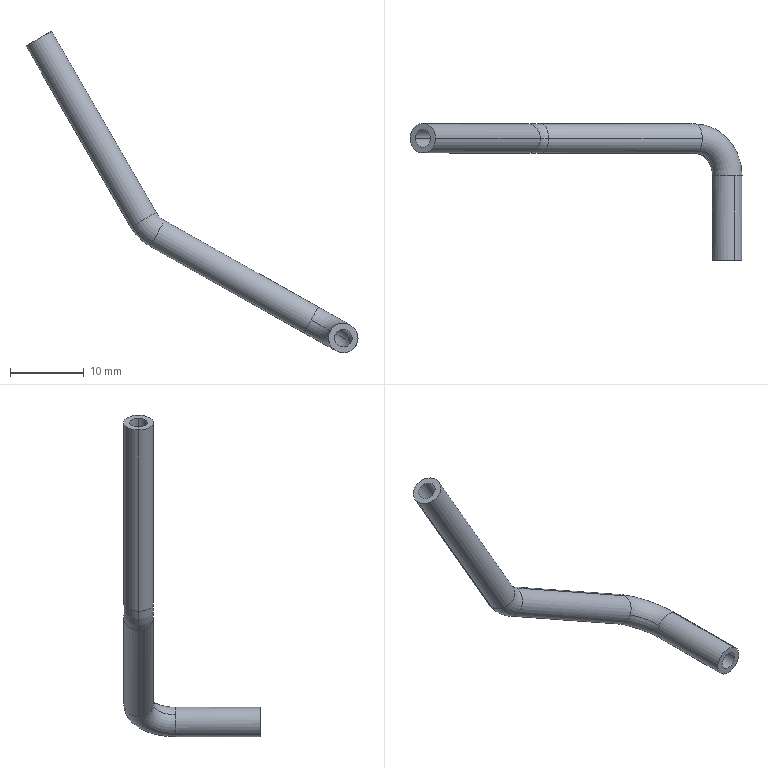Component | SolidWorks | WaterPipe2-1 | 1 solid | 22 faces | box 44.91 x 18.45 x 43.5 mm | volume 596 mm3 | cylinder 12 | torus 8 | plane 2 | commonest cylinder face diameters 2.4 x6 4 x6
build123d program:
from build123d import *

# Parameters (mm, degrees)
SCAN_THIN_FEATURE1_PROFILE_R   = 2
SCAN_THIN_FEATURE1_PROFILE_R_2 = 1.2


with BuildPart() as part:
    # Scan-Thin Feature1: sweep along a curve in space
    with BuildLine() as scan_thin_feature1_path:
        Line((0, -15.405, 0), (0, -3.951, 0))
        ThreePointArc((-5, 1.049, 0), (-1.464, -0.4154, 0), (0, -3.951, 0))
        Line((-5, 1.049, 0), (-28.841, 1.049, 0))
        ThreePointArc((-31.391, 1.049, 0.6989), (-30.163, 1.049, 0.1779), (-28.841, 1.049, 0))
        Line((-31.391, 1.049, 0.6989), (-55.737, 1.049, 15.131))
    # Scan-Thin Feature1 profile (on start of the path) → Scan-Thin Feature1 (sweep)
    with BuildSketch(Plane.ZX.offset(-15.405)):
        Circle(SCAN_THIN_FEATURE1_PROFILE_R)
        Circle(SCAN_THIN_FEATURE1_PROFILE_R_2, mode=Mode.SUBTRACT)
    sweep(path=scan_thin_feature1_path.line)


solid = part.part

# Placed as in the assembly
solid = solid.moved(Location((-15.981, 32.512, 80), (0, 29.34, 0)))
STEP:
#1=COLOUR_RGB('',0.7922,0.8196,0.9333);
#2=FILL_AREA_STYLE_COLOUR('',#1);
#3=FILL_AREA_STYLE('',(#2));
#4=SURFACE_STYLE_FILL_AREA(#3);
#5=SURFACE_SIDE_STYLE('',(#4));
#6=SURFACE_STYLE_USAGE(.BOTH.,#5);
#7=PRESENTATION_STYLE_ASSIGNMENT((#6));
#8=CARTESIAN_POINT('',(-1.596,1.321,3.747));
#9=VERTEX_POINT('',#8);
#10=CARTESIAN_POINT('',(-1.642,1.321,3.665));
#11=VERTEX_POINT('',#10);
#12=CARTESIAN_POINT('',(-1.619,1.321,3.706));
#13=DIRECTION('',(0.8717,-0.,-0.49));
#14=DIRECTION('',(0.49,-0.,0.8717));
#15=AXIS2_PLACEMENT_3D('',#12,#13,#14);
#16=CIRCLE('',#15,0.04724);
#17=EDGE_CURVE('',#9,#11,#16,.T.);
#18=ORIENTED_EDGE('',*,*,#17,.T.);
#19=CARTESIAN_POINT('',(-1.734,1.321,3.756));
#20=VERTEX_POINT('',#19);
#21=CARTESIAN_POINT('',(-1.523,1.321,3.878));
#22=DIRECTION('',(-0.,1.,-0.));
#23=DIRECTION('',(0.,0.,1.));
#24=AXIS2_PLACEMENT_3D('',#21,#22,#23);
#25=CIRCLE('',#24,0.2441);
#26=EDGE_CURVE('',#11,#20,#25,.T.);
#27=ORIENTED_EDGE('',*,*,#26,.T.);
#28=CARTESIAN_POINT('',(-1.652,1.321,3.803));
#29=VERTEX_POINT('',#28);
#30=CARTESIAN_POINT('',(-1.693,1.321,3.779));
#31=DIRECTION('',(0.5,-0.,-0.866));
#32=DIRECTION('',(-0.866,0.,-0.5));
#33=AXIS2_PLACEMENT_3D('',#30,#31,#32);
#34=CIRCLE('',#33,0.04724);
#35=EDGE_CURVE('',#29,#20,#34,.T.);
#36=ORIENTED_EDGE('',*,*,#35,.F.);
#37=CARTESIAN_POINT('',(-1.523,1.321,3.878));
#38=DIRECTION('',(-0.,1.,-0.));
#39=DIRECTION('',(0.,0.,1.));
#40=AXIS2_PLACEMENT_3D('',#37,#38,#39);
#41=CIRCLE('',#40,0.1496);
#42=EDGE_CURVE('',#9,#29,#41,.T.);
#43=ORIENTED_EDGE('',*,*,#42,.F.);
#44=EDGE_LOOP('',(#18,#27,#36,#43));
#45=FACE_OUTER_BOUND('',#44,.T.);
#46=CARTESIAN_POINT('',(-1.523,1.321,3.878));
#47=DIRECTION('',(-0.,1.,-0.));
#48=DIRECTION('',(0.49,0.,0.8717));
#49=AXIS2_PLACEMENT_3D('',#46,#47,#48);
#50=TOROIDAL_SURFACE('',#49,0.1969,0.04724);
#51=ADVANCED_FACE('',(#45),#50,.F.);
#52=CARTESIAN_POINT('',(-0.6523,1.124,3.108));
#53=VERTEX_POINT('',#52);
#54=CARTESIAN_POINT('',(-0.588,1.124,3.126));
#55=VERTEX_POINT('',#54);
#56=CARTESIAN_POINT('',(-0.6292,1.124,3.15));
#57=DIRECTION('',(0.,-1.,0.));
#58=DIRECTION('',(0.49,0.,0.8717));
#59=AXIS2_PLACEMENT_3D('',#56,#57,#58);
#60=CIRCLE('',#59,0.04724);
#61=EDGE_CURVE('',#53,#55,#60,.T.);
#62=ORIENTED_EDGE('',*,*,#61,.T.);
#63=CARTESIAN_POINT('',(-0.8008,1.369,3.246));
#64=VERTEX_POINT('',#63);
#65=CARTESIAN_POINT('',(-0.8008,1.124,3.246));
#66=DIRECTION('',(0.49,0.,0.8717));
#67=DIRECTION('',(0.8717,0.,-0.49));
#68=AXIS2_PLACEMENT_3D('',#65,#66,#67);
#69=CIRCLE('',#68,0.2441);
#70=EDGE_CURVE('',#55,#64,#69,.T.);
#71=ORIENTED_EDGE('',*,*,#70,.T.);
#72=CARTESIAN_POINT('',(-0.8239,1.321,3.205));
#73=VERTEX_POINT('',#72);
#74=CARTESIAN_POINT('',(-0.8008,1.321,3.246));
#75=DIRECTION('',(0.8717,0.,-0.49));
#76=DIRECTION('',(-0.,1.,0.));
#77=AXIS2_PLACEMENT_3D('',#74,#75,#76);
#78=CIRCLE('',#77,0.04724);
#79=EDGE_CURVE('',#73,#64,#78,.T.);
#80=ORIENTED_EDGE('',*,*,#79,.F.);
#81=CARTESIAN_POINT('',(-0.8008,1.274,3.246));
#82=VERTEX_POINT('',#81);
#83=CARTESIAN_POINT('',(-0.8008,1.321,3.246));
#84=DIRECTION('',(0.8717,0.,-0.49));
#85=DIRECTION('',(-0.,1.,0.));
#86=AXIS2_PLACEMENT_3D('',#83,#84,#85);
#87=CIRCLE('',#86,0.04724);
#88=EDGE_CURVE('',#82,#73,#87,.T.);
#89=ORIENTED_EDGE('',*,*,#88,.F.);
#90=CARTESIAN_POINT('',(-0.6704,1.124,3.173));
#91=VERTEX_POINT('',#90);
#92=CARTESIAN_POINT('',(-0.8008,1.124,3.246));
#93=DIRECTION('',(0.49,0.,0.8717));
#94=DIRECTION('',(0.8717,0.,-0.49));
#95=AXIS2_PLACEMENT_3D('',#92,#93,#94);
#96=CIRCLE('',#95,0.1496);
#97=EDGE_CURVE('',#91,#82,#96,.T.);
#98=ORIENTED_EDGE('',*,*,#97,.F.);
#99=CARTESIAN_POINT('',(-0.6292,1.124,3.15));
#100=DIRECTION('',(0.,-1.,0.));
#101=DIRECTION('',(0.49,0.,0.8717));
#102=AXIS2_PLACEMENT_3D('',#99,#100,#101);
#103=CIRCLE('',#102,0.04724);
#104=EDGE_CURVE('',#91,#53,#103,.T.);
#105=ORIENTED_EDGE('',*,*,#104,.T.);
#106=EDGE_LOOP('',(#62,#71,#80,#89,#98,#105));
#107=FACE_OUTER_BOUND('',#106,.T.);
#108=CARTESIAN_POINT('',(-0.8008,1.124,3.246));
#109=DIRECTION('',(0.49,0.,0.8717));
#110=DIRECTION('',(0.8717,0.,-0.49));
#111=AXIS2_PLACEMENT_3D('',#108,#109,#110);
#112=TOROIDAL_SURFACE('',#111,0.1969,0.04724);
#113=ADVANCED_FACE('',(#107),#112,.F.);
#114=CARTESIAN_POINT('',(-1.658,1.321,3.637));
#115=VERTEX_POINT('',#114);
#116=CARTESIAN_POINT('',(-1.58,1.321,3.775));
#117=VERTEX_POINT('',#116);
#118=CARTESIAN_POINT('',(-1.619,1.321,3.706));
#119=DIRECTION('',(0.8717,-0.,-0.49));
#120=DIRECTION('',(-0.49,0.,-0.8717));
#121=AXIS2_PLACEMENT_3D('',#118,#119,#120);
#122=CIRCLE('',#121,0.07874);
#123=EDGE_CURVE('',#115,#117,#122,.T.);
#124=ORIENTED_EDGE('',*,*,#123,.F.);
#125=CARTESIAN_POINT('',(-1.761,1.321,3.74));
#126=VERTEX_POINT('',#125);
#127=CARTESIAN_POINT('',(-1.523,1.321,3.878));
#128=DIRECTION('',(-0.,1.,-0.));
#129=DIRECTION('',(0.,0.,1.));
#130=AXIS2_PLACEMENT_3D('',#127,#128,#129);
#131=CIRCLE('',#130,0.2756);
#132=EDGE_CURVE('',#115,#126,#131,.T.);
#133=ORIENTED_EDGE('',*,*,#132,.T.);
#134=CARTESIAN_POINT('',(-1.625,1.321,3.819));
#135=VERTEX_POINT('',#134);
#136=CARTESIAN_POINT('',(-1.693,1.321,3.779));
#137=DIRECTION('',(0.5,-0.,-0.866));
#138=DIRECTION('',(-0.866,0.,-0.5));
#139=AXIS2_PLACEMENT_3D('',#136,#137,#138);
#140=CIRCLE('',#139,0.07874);
#141=EDGE_CURVE('',#126,#135,#140,.T.);
#142=ORIENTED_EDGE('',*,*,#141,.T.);
#143=CARTESIAN_POINT('',(-1.523,1.321,3.878));
#144=DIRECTION('',(-0.,1.,-0.));
#145=DIRECTION('',(0.,0.,1.));
#146=AXIS2_PLACEMENT_3D('',#143,#144,#145);
#147=CIRCLE('',#146,0.1181);
#148=EDGE_CURVE('',#117,#135,#147,.T.);
#149=ORIENTED_EDGE('',*,*,#148,.F.);
#150=EDGE_LOOP('',(#124,#133,#142,#149));
#151=FACE_OUTER_BOUND('',#150,.T.);
#152=CARTESIAN_POINT('',(-1.523,1.321,3.878));
#153=DIRECTION('',(-0.,1.,-0.));
#154=DIRECTION('',(0.49,0.,0.8717));
#155=AXIS2_PLACEMENT_3D('',#152,#153,#154);
#156=TOROIDAL_SURFACE('',#155,0.1969,0.07874);
#157=ADVANCED_FACE('',(#151),#156,.T.);
#158=CARTESIAN_POINT('',(-0.5605,1.124,3.111));
#159=VERTEX_POINT('',#158);
#160=CARTESIAN_POINT('',(-0.5906,1.124,3.218));
#161=VERTEX_POINT('',#160);
#162=CARTESIAN_POINT('',(-0.6292,1.124,3.15));
#163=DIRECTION('',(-0.,-1.,-0.));
#164=DIRECTION('',(-0.49,0.,-0.8717));
#165=AXIS2_PLACEMENT_3D('',#162,#163,#164);
#166=CIRCLE('',#165,0.07874);
#167=EDGE_CURVE('',#159,#161,#166,.T.);
#168=ORIENTED_EDGE('',*,*,#167,.F.);
#169=CARTESIAN_POINT('',(-0.8008,1.4,3.246));
#170=VERTEX_POINT('',#169);
#171=CARTESIAN_POINT('',(-0.8008,1.124,3.246));
#172=DIRECTION('',(0.49,0.,0.8717));
#173=DIRECTION('',(0.8717,0.,-0.49));
#174=AXIS2_PLACEMENT_3D('',#171,#172,#173);
#175=CIRCLE('',#174,0.2756);
#176=EDGE_CURVE('',#159,#170,#175,.T.);
#177=ORIENTED_EDGE('',*,*,#176,.T.);
#178=CARTESIAN_POINT('',(-0.7622,1.321,3.315));
#179=VERTEX_POINT('',#178);
#180=CARTESIAN_POINT('',(-0.8008,1.321,3.246));
#181=DIRECTION('',(0.8717,-0.,-0.49));
#182=DIRECTION('',(-0.49,0.,-0.8717));
#183=AXIS2_PLACEMENT_3D('',#180,#181,#182);
#184=CIRCLE('',#183,0.07874);
#185=EDGE_CURVE('',#170,#179,#184,.T.);
#186=ORIENTED_EDGE('',*,*,#185,.T.);
#187=CARTESIAN_POINT('',(-0.8008,1.243,3.246));
#188=VERTEX_POINT('',#187);
#189=CARTESIAN_POINT('',(-0.8008,1.321,3.246));
#190=DIRECTION('',(0.8717,-0.,-0.49));
#191=DIRECTION('',(-0.49,0.,-0.8717));
#192=AXIS2_PLACEMENT_3D('',#189,#190,#191);
#193=CIRCLE('',#192,0.07874);
#194=EDGE_CURVE('',#179,#188,#193,.T.);
#195=ORIENTED_EDGE('',*,*,#194,.T.);
#196=CARTESIAN_POINT('',(-0.6978,1.124,3.188));
#197=VERTEX_POINT('',#196);
#198=CARTESIAN_POINT('',(-0.8008,1.124,3.246));
#199=DIRECTION('',(0.49,0.,0.8717));
#200=DIRECTION('',(0.8717,0.,-0.49));
#201=AXIS2_PLACEMENT_3D('',#198,#199,#200);
#202=CIRCLE('',#201,0.1181);
#203=EDGE_CURVE('',#197,#188,#202,.T.);
#204=ORIENTED_EDGE('',*,*,#203,.F.);
#205=CARTESIAN_POINT('',(-0.6292,1.124,3.15));
#206=DIRECTION('',(-0.,-1.,-0.));
#207=DIRECTION('',(-0.49,0.,-0.8717));
#208=AXIS2_PLACEMENT_3D('',#205,#206,#207);
#209=CIRCLE('',#208,0.07874);
#210=EDGE_CURVE('',#161,#197,#209,.T.);
#211=ORIENTED_EDGE('',*,*,#210,.F.);
#212=EDGE_LOOP('',(#168,#177,#186,#195,#204,#211));
#213=FACE_OUTER_BOUND('',#212,.T.);
#214=CARTESIAN_POINT('',(-0.8008,1.124,3.246));
#215=DIRECTION('',(0.49,0.,0.8717));
#216=DIRECTION('',(0.8717,0.,-0.49));
#217=AXIS2_PLACEMENT_3D('',#214,#215,#216);
#218=TOROIDAL_SURFACE('',#217,0.1969,0.07874);
#219=ADVANCED_FACE('',(#213),#218,.T.);
#220=ORIENTED_EDGE('',*,*,#35,.T.);
#221=CARTESIAN_POINT('',(-2.291,1.321,4.721));
#222=VERTEX_POINT('',#221);
#223=CARTESIAN_POINT('',(-1.734,1.321,3.756));
#224=DIRECTION('',(-0.5,0.,0.866));
#225=VECTOR('',#224,39.37);
#226=LINE('',#223,#225);
#227=EDGE_CURVE('',#20,#222,#226,.T.);
#228=ORIENTED_EDGE('',*,*,#227,.T.);
#229=CARTESIAN_POINT('',(-2.209,1.321,4.768));
#230=VERTEX_POINT('',#229);
#231=CARTESIAN_POINT('',(-2.25,1.321,4.744));
#232=DIRECTION('',(0.5,-0.,-0.866));
#233=DIRECTION('',(-0.866,0.,-0.5));
#234=AXIS2_PLACEMENT_3D('',#231,#232,#233);
#235=CIRCLE('',#234,0.04724);
#236=EDGE_CURVE('',#230,#222,#235,.T.);
#237=ORIENTED_EDGE('',*,*,#236,.F.);
#238=CARTESIAN_POINT('',(-1.652,1.321,3.803));
#239=DIRECTION('',(-0.5,0.,0.866));
#240=VECTOR('',#239,39.37);
#241=LINE('',#238,#240);
#242=EDGE_CURVE('',#29,#230,#241,.T.);
#243=ORIENTED_EDGE('',*,*,#242,.F.);
#244=EDGE_LOOP('',(#220,#228,#237,#243));
#245=FACE_OUTER_BOUND('',#244,.T.);
#246=CARTESIAN_POINT('',(-1.693,1.321,3.779));
#247=DIRECTION('',(-0.5,0.,0.866));
#248=DIRECTION('',(0.866,0.,0.5));
#249=AXIS2_PLACEMENT_3D('',#246,#247,#248);
#250=CYLINDRICAL_SURFACE('',#249,0.04724);
#251=ADVANCED_FACE('',(#245),#250,.F.);
#252=CARTESIAN_POINT('',(-0.7776,1.321,3.287));
#253=VERTEX_POINT('',#252);
#254=CARTESIAN_POINT('',(-0.8008,1.321,3.246));
#255=DIRECTION('',(0.8717,0.,-0.49));
#256=DIRECTION('',(-0.,1.,0.));
#257=AXIS2_PLACEMENT_3D('',#254,#255,#256);
#258=CIRCLE('',#257,0.04724);
#259=EDGE_CURVE('',#253,#82,#258,.T.);
#260=ORIENTED_EDGE('',*,*,#259,.T.);
#261=ORIENTED_EDGE('',*,*,#88,.T.);
#262=CARTESIAN_POINT('',(-0.8239,1.321,3.205));
#263=DIRECTION('',(-0.8717,0.,0.49));
#264=VECTOR('',#263,39.37);
#265=LINE('',#262,#264);
#266=EDGE_CURVE('',#73,#11,#265,.T.);
#267=ORIENTED_EDGE('',*,*,#266,.T.);
#268=ORIENTED_EDGE('',*,*,#17,.F.);
#269=CARTESIAN_POINT('',(-0.7776,1.321,3.287));
#270=DIRECTION('',(-0.8717,0.,0.49));
#271=VECTOR('',#270,39.37);
#272=LINE('',#269,#271);
#273=EDGE_CURVE('',#253,#9,#272,.T.);
#274=ORIENTED_EDGE('',*,*,#273,.F.);
#275=EDGE_LOOP('',(#260,#261,#267,#268,#274));
#276=FACE_OUTER_BOUND('',#275,.T.);
#277=CARTESIAN_POINT('',(-0.8008,1.321,3.246));
#278=DIRECTION('',(-0.8717,0.,0.49));
#279=DIRECTION('',(0.49,0.,0.8717));
#280=AXIS2_PLACEMENT_3D('',#277,#278,#279);
#281=CYLINDRICAL_SURFACE('',#280,0.04724);
#282=ADVANCED_FACE('',(#276),#281,.F.);
#283=CARTESIAN_POINT('',(-0.606,0.6735,3.191));
#284=VERTEX_POINT('',#283);
#285=CARTESIAN_POINT('',(-0.6523,0.6735,3.108));
#286=VERTEX_POINT('',#285);
#287=CARTESIAN_POINT('',(-0.6292,0.6735,3.15));
#288=DIRECTION('',(-0.,-1.,-0.));
#289=DIRECTION('',(-0.49,0.,-0.8717));
#290=AXIS2_PLACEMENT_3D('',#287,#288,#289);
#291=CIRCLE('',#290,0.04724);
#292=EDGE_CURVE('',#284,#286,#291,.T.);
#293=ORIENTED_EDGE('',*,*,#292,.T.);
#294=CARTESIAN_POINT('',(-0.6523,0.6735,3.108));
#295=DIRECTION('',(-0.,1.,-0.));
#296=VECTOR('',#295,39.37);
#297=LINE('',#294,#296);
#298=EDGE_CURVE('',#286,#53,#297,.T.);
#299=ORIENTED_EDGE('',*,*,#298,.T.);
#300=ORIENTED_EDGE('',*,*,#104,.F.);
#301=CARTESIAN_POINT('',(-0.606,1.124,3.191));
#302=VERTEX_POINT('',#301);
#303=CARTESIAN_POINT('',(-0.6292,1.124,3.15));
#304=DIRECTION('',(0.,-1.,0.));
#305=DIRECTION('',(0.49,0.,0.8717));
#306=AXIS2_PLACEMENT_3D('',#303,#304,#305);
#307=CIRCLE('',#306,0.04724);
#308=EDGE_CURVE('',#302,#91,#307,.T.);
#309=ORIENTED_EDGE('',*,*,#308,.F.);
#310=CARTESIAN_POINT('',(-0.606,0.6735,3.191));
#311=DIRECTION('',(-0.,1.,-0.));
#312=VECTOR('',#311,39.37);
#313=LINE('',#310,#312);
#314=EDGE_CURVE('',#284,#302,#313,.T.);
#315=ORIENTED_EDGE('',*,*,#314,.F.);
#316=EDGE_LOOP('',(#293,#299,#300,#309,#315));
#317=FACE_OUTER_BOUND('',#316,.T.);
#318=CARTESIAN_POINT('',(-0.6292,0.6735,3.15));
#319=DIRECTION('',(-0.,1.,-0.));
#320=DIRECTION('',(0.49,0.,0.8717));
#321=AXIS2_PLACEMENT_3D('',#318,#319,#320);
#322=CYLINDRICAL_SURFACE('',#321,0.04724);
#323=ADVANCED_FACE('',(#317),#322,.F.);
#324=ORIENTED_EDGE('',*,*,#141,.F.);
#325=CARTESIAN_POINT('',(-2.318,1.321,4.705));
#326=VERTEX_POINT('',#325);
#327=CARTESIAN_POINT('',(-1.761,1.321,3.74));
#328=DIRECTION('',(-0.5,0.,0.866));
#329=VECTOR('',#328,39.37);
#330=LINE('',#327,#329);
#331=EDGE_CURVE('',#126,#326,#330,.T.);
#332=ORIENTED_EDGE('',*,*,#331,.T.);
#333=CARTESIAN_POINT('',(-2.182,1.321,4.784));
#334=VERTEX_POINT('',#333);
#335=CARTESIAN_POINT('',(-2.25,1.321,4.744));
#336=DIRECTION('',(0.5,-0.,-0.866));
#337=DIRECTION('',(-0.866,0.,-0.5));
#338=AXIS2_PLACEMENT_3D('',#335,#336,#337);
#339=CIRCLE('',#338,0.07874);
#340=EDGE_CURVE('',#326,#334,#339,.T.);
#341=ORIENTED_EDGE('',*,*,#340,.T.);
#342=CARTESIAN_POINT('',(-1.625,1.321,3.819));
#343=DIRECTION('',(-0.5,0.,0.866));
#344=VECTOR('',#343,39.37);
#345=LINE('',#342,#344);
#346=EDGE_CURVE('',#135,#334,#345,.T.);
#347=ORIENTED_EDGE('',*,*,#346,.F.);
#348=EDGE_LOOP('',(#324,#332,#341,#347));
#349=FACE_OUTER_BOUND('',#348,.T.);
#350=CARTESIAN_POINT('',(-1.693,1.321,3.779));
#351=DIRECTION('',(-0.5,0.,0.866));
#352=DIRECTION('',(0.866,0.,0.5));
#353=AXIS2_PLACEMENT_3D('',#350,#351,#352);
#354=CYLINDRICAL_SURFACE('',#353,0.07874);
#355=ADVANCED_FACE('',(#349),#354,.T.);
#356=CARTESIAN_POINT('',(-0.8394,1.321,3.177));
#357=VERTEX_POINT('',#356);
#358=CARTESIAN_POINT('',(-0.8008,1.321,3.246));
#359=DIRECTION('',(0.8717,-0.,-0.49));
#360=DIRECTION('',(-0.49,0.,-0.8717));
#361=AXIS2_PLACEMENT_3D('',#358,#359,#360);
#362=CIRCLE('',#361,0.07874);
#363=EDGE_CURVE('',#357,#170,#362,.T.);
#364=ORIENTED_EDGE('',*,*,#363,.F.);
#365=CARTESIAN_POINT('',(-0.8394,1.321,3.177));
#366=DIRECTION('',(-0.8717,0.,0.49));
#367=VECTOR('',#366,39.37);
#368=LINE('',#365,#367);
#369=EDGE_CURVE('',#357,#115,#368,.T.);
#370=ORIENTED_EDGE('',*,*,#369,.T.);
#371=ORIENTED_EDGE('',*,*,#123,.T.);
#372=CARTESIAN_POINT('',(-0.7622,1.321,3.315));
#373=DIRECTION('',(-0.8717,0.,0.49));
#374=VECTOR('',#373,39.37);
#375=LINE('',#372,#374);
#376=EDGE_CURVE('',#179,#117,#375,.T.);
#377=ORIENTED_EDGE('',*,*,#376,.F.);
#378=ORIENTED_EDGE('',*,*,#185,.F.);
#379=EDGE_LOOP('',(#364,#370,#371,#377,#378));
#380=FACE_OUTER_BOUND('',#379,.T.);
#381=CARTESIAN_POINT('',(-0.8008,1.321,3.246));
#382=DIRECTION('',(-0.8717,0.,0.49));
#383=DIRECTION('',(0.49,0.,0.8717));
#384=AXIS2_PLACEMENT_3D('',#381,#382,#383);
#385=CYLINDRICAL_SURFACE('',#384,0.07874);
#386=ADVANCED_FACE('',(#380),#385,.T.);
#387=CARTESIAN_POINT('',(-0.6678,0.6735,3.081));
#388=VERTEX_POINT('',#387);
#389=CARTESIAN_POINT('',(-0.5906,0.6735,3.218));
#390=VERTEX_POINT('',#389);
#391=CARTESIAN_POINT('',(-0.6292,0.6735,3.15));
#392=DIRECTION('',(-0.,-1.,-0.));
#393=DIRECTION('',(-0.49,0.,-0.8717));
#394=AXIS2_PLACEMENT_3D('',#391,#392,#393);
#395=CIRCLE('',#394,0.07874);
#396=EDGE_CURVE('',#388,#390,#395,.T.);
#397=ORIENTED_EDGE('',*,*,#396,.F.);
#398=CARTESIAN_POINT('',(-0.6678,1.124,3.081));
#399=VERTEX_POINT('',#398);
#400=CARTESIAN_POINT('',(-0.6678,0.6735,3.081));
#401=DIRECTION('',(-0.,1.,-0.));
#402=VECTOR('',#401,39.37);
#403=LINE('',#400,#402);
#404=EDGE_CURVE('',#388,#399,#403,.T.);
#405=ORIENTED_EDGE('',*,*,#404,.T.);
#406=CARTESIAN_POINT('',(-0.6292,1.124,3.15));
#407=DIRECTION('',(-0.,-1.,-0.));
#408=DIRECTION('',(-0.49,0.,-0.8717));
#409=AXIS2_PLACEMENT_3D('',#406,#407,#408);
#410=CIRCLE('',#409,0.07874);
#411=EDGE_CURVE('',#399,#159,#410,.T.);
#412=ORIENTED_EDGE('',*,*,#411,.T.);
#413=ORIENTED_EDGE('',*,*,#167,.T.);
#414=CARTESIAN_POINT('',(-0.5906,0.6735,3.218));
#415=DIRECTION('',(-0.,1.,-0.));
#416=VECTOR('',#415,39.37);
#417=LINE('',#414,#416);
#418=EDGE_CURVE('',#390,#161,#417,.T.);
#419=ORIENTED_EDGE('',*,*,#418,.F.);
#420=EDGE_LOOP('',(#397,#405,#412,#413,#419));
#421=FACE_OUTER_BOUND('',#420,.T.);
#422=CARTESIAN_POINT('',(-0.6292,0.6735,3.15));
#423=DIRECTION('',(-0.,1.,-0.));
#424=DIRECTION('',(0.49,0.,0.8717));
#425=AXIS2_PLACEMENT_3D('',#422,#423,#424);
#426=CYLINDRICAL_SURFACE('',#425,0.07874);
#427=ADVANCED_FACE('',(#421),#426,.T.);
#428=ORIENTED_EDGE('',*,*,#331,.F.);
#429=CARTESIAN_POINT('',(-1.693,1.321,3.779));
#430=DIRECTION('',(0.5,-0.,-0.866));
#431=DIRECTION('',(-0.866,0.,-0.5));
#432=AXIS2_PLACEMENT_3D('',#429,#430,#431);
#433=CIRCLE('',#432,0.07874);
#434=EDGE_CURVE('',#135,#126,#433,.T.);
#435=ORIENTED_EDGE('',*,*,#434,.F.);
#436=ORIENTED_EDGE('',*,*,#346,.T.);
#437=CARTESIAN_POINT('',(-2.25,1.321,4.744));
#438=DIRECTION('',(0.5,-0.,-0.866));
#439=DIRECTION('',(-0.866,0.,-0.5));
#440=AXIS2_PLACEMENT_3D('',#437,#438,#439);
#441=CIRCLE('',#440,0.07874);
#442=EDGE_CURVE('',#334,#326,#441,.T.);
#443=ORIENTED_EDGE('',*,*,#442,.T.);
#444=EDGE_LOOP('',(#428,#435,#436,#443));
#445=FACE_OUTER_BOUND('',#444,.T.);
#446=CARTESIAN_POINT('',(-1.693,1.321,3.779));
#447=DIRECTION('',(-0.5,0.,0.866));
#448=DIRECTION('',(0.866,0.,0.5));
#449=AXIS2_PLACEMENT_3D('',#446,#447,#448);
#450=CYLINDRICAL_SURFACE('',#449,0.07874);
#451=ADVANCED_FACE('',(#445),#450,.T.);
#452=ORIENTED_EDGE('',*,*,#132,.F.);
#453=CARTESIAN_POINT('',(-1.619,1.321,3.706));
#454=DIRECTION('',(0.8717,-0.,-0.49));
#455=DIRECTION('',(-0.49,0.,-0.8717));
#456=AXIS2_PLACEMENT_3D('',#453,#454,#455);
#457=CIRCLE('',#456,0.07874);
#458=EDGE_CURVE('',#117,#115,#457,.T.);
#459=ORIENTED_EDGE('',*,*,#458,.F.);
#460=ORIENTED_EDGE('',*,*,#148,.T.);
#461=ORIENTED_EDGE('',*,*,#434,.T.);
#462=EDGE_LOOP('',(#452,#459,#460,#461));
#463=FACE_OUTER_BOUND('',#462,.T.);
#464=CARTESIAN_POINT('',(-1.523,1.321,3.878));
#465=DIRECTION('',(-0.,1.,-0.));
#466=DIRECTION('',(0.49,0.,0.8717));
#467=AXIS2_PLACEMENT_3D('',#464,#465,#466);
#468=TOROIDAL_SURFACE('',#467,0.1969,0.07874);
#469=ADVANCED_FACE('',(#463),#468,.T.);
#470=ORIENTED_EDGE('',*,*,#369,.F.);
#471=CARTESIAN_POINT('',(-0.8008,1.321,3.246));
#472=DIRECTION('',(0.8717,-0.,-0.49));
#473=DIRECTION('',(-0.49,0.,-0.8717));
#474=AXIS2_PLACEMENT_3D('',#471,#472,#473);
#475=CIRCLE('',#474,0.07874);
#476=EDGE_CURVE('',#188,#357,#475,.T.);
#477=ORIENTED_EDGE('',*,*,#476,.F.);
#478=ORIENTED_EDGE('',*,*,#194,.F.);
#479=ORIENTED_EDGE('',*,*,#376,.T.);
#480=ORIENTED_EDGE('',*,*,#458,.T.);
#481=EDGE_LOOP('',(#470,#477,#478,#479,#480));
#482=FACE_OUTER_BOUND('',#481,.T.);
#483=CARTESIAN_POINT('',(-0.8008,1.321,3.246));
#484=DIRECTION('',(-0.8717,0.,0.49));
#485=DIRECTION('',(0.49,0.,0.8717));
#486=AXIS2_PLACEMENT_3D('',#483,#484,#485);
#487=CYLINDRICAL_SURFACE('',#486,0.07874);
#488=ADVANCED_FACE('',(#482),#487,.T.);
#489=ORIENTED_EDGE('',*,*,#176,.F.);
#490=ORIENTED_EDGE('',*,*,#411,.F.);
#491=CARTESIAN_POINT('',(-0.6292,1.124,3.15));
#492=DIRECTION('',(-0.,-1.,-0.));
#493=DIRECTION('',(-0.49,0.,-0.8717));
#494=AXIS2_PLACEMENT_3D('',#491,#492,#493);
#495=CIRCLE('',#494,0.07874);
#496=EDGE_CURVE('',#197,#399,#495,.T.);
#497=ORIENTED_EDGE('',*,*,#496,.F.);
#498=ORIENTED_EDGE('',*,*,#203,.T.);
#499=ORIENTED_EDGE('',*,*,#476,.T.);
#500=ORIENTED_EDGE('',*,*,#363,.T.);
#501=EDGE_LOOP('',(#489,#490,#497,#498,#499,#500));
#502=FACE_OUTER_BOUND('',#501,.T.);
#503=CARTESIAN_POINT('',(-0.8008,1.124,3.246));
#504=DIRECTION('',(0.49,0.,0.8717));
#505=DIRECTION('',(0.8717,0.,-0.49));
#506=AXIS2_PLACEMENT_3D('',#503,#504,#505);
#507=TOROIDAL_SURFACE('',#506,0.1969,0.07874);
#508=ADVANCED_FACE('',(#502),#507,.T.);
#509=ORIENTED_EDGE('',*,*,#404,.F.);
#510=CARTESIAN_POINT('',(-0.6292,0.6735,3.15));
#511=DIRECTION('',(-0.,-1.,-0.));
#512=DIRECTION('',(-0.49,0.,-0.8717));
#513=AXIS2_PLACEMENT_3D('',#510,#511,#512);
#514=CIRCLE('',#513,0.07874);
#515=EDGE_CURVE('',#390,#388,#514,.T.);
#516=ORIENTED_EDGE('',*,*,#515,.F.);
#517=ORIENTED_EDGE('',*,*,#418,.T.);
#518=ORIENTED_EDGE('',*,*,#210,.T.);
#519=ORIENTED_EDGE('',*,*,#496,.T.);
#520=EDGE_LOOP('',(#509,#516,#517,#518,#519));
#521=FACE_OUTER_BOUND('',#520,.T.);
#522=CARTESIAN_POINT('',(-0.6292,0.6735,3.15));
#523=DIRECTION('',(-0.,1.,-0.));
#524=DIRECTION('',(0.49,0.,0.8717));
#525=AXIS2_PLACEMENT_3D('',#522,#523,#524);
#526=CYLINDRICAL_SURFACE('',#525,0.07874);
#527=ADVANCED_FACE('',(#521),#526,.T.);
#528=ORIENTED_EDGE('',*,*,#236,.T.);
#529=CARTESIAN_POINT('',(-2.25,1.321,4.744));
#530=DIRECTION('',(0.5,-0.,-0.866));
#531=DIRECTION('',(-0.866,0.,-0.5));
#532=AXIS2_PLACEMENT_3D('',#529,#530,#531);
#533=CIRCLE('',#532,0.04724);
#534=EDGE_CURVE('',#222,#230,#533,.T.);
#535=ORIENTED_EDGE('',*,*,#534,.T.);
#536=EDGE_LOOP('',(#528,#535));
#537=FACE_BOUND('',#536,.T.);
#538=ORIENTED_EDGE('',*,*,#442,.F.);
#539=ORIENTED_EDGE('',*,*,#340,.F.);
#540=EDGE_LOOP('',(#538,#539));
#541=FACE_OUTER_BOUND('',#540,.T.);
#542=CARTESIAN_POINT('',(-2.25,1.321,4.744));
#543=DIRECTION('',(0.5,-0.,-0.866));
#544=DIRECTION('',(-0.866,-0.,-0.5));
#545=AXIS2_PLACEMENT_3D('',#542,#543,#544);
#546=PLANE('',#545);
#547=ADVANCED_FACE('',(#537,#541),#546,.F.);
#548=ORIENTED_EDGE('',*,*,#292,.F.);
#549=CARTESIAN_POINT('',(-0.6292,0.6735,3.15));
#550=DIRECTION('',(-0.,-1.,-0.));
#551=DIRECTION('',(-0.49,0.,-0.8717));
#552=AXIS2_PLACEMENT_3D('',#549,#550,#551);
#553=CIRCLE('',#552,0.04724);
#554=EDGE_CURVE('',#286,#284,#553,.T.);
#555=ORIENTED_EDGE('',*,*,#554,.F.);
#556=EDGE_LOOP('',(#548,#555));
#557=FACE_BOUND('',#556,.T.);
#558=ORIENTED_EDGE('',*,*,#515,.T.);
#559=ORIENTED_EDGE('',*,*,#396,.T.);
#560=EDGE_LOOP('',(#558,#559));
#561=FACE_OUTER_BOUND('',#560,.T.);
#562=CARTESIAN_POINT('',(-0.6292,0.6735,3.15));
#563=DIRECTION('',(-0.,-1.,-0.));
#564=DIRECTION('',(-0.49,0.,-0.8717));
#565=AXIS2_PLACEMENT_3D('',#562,#563,#564);
#566=PLANE('',#565);
#567=ADVANCED_FACE('',(#557,#561),#566,.T.);
#568=ORIENTED_EDGE('',*,*,#227,.F.);
#569=CARTESIAN_POINT('',(-1.693,1.321,3.779));
#570=DIRECTION('',(0.5,-0.,-0.866));
#571=DIRECTION('',(-0.866,0.,-0.5));
#572=AXIS2_PLACEMENT_3D('',#569,#570,#571);
#573=CIRCLE('',#572,0.04724);
#574=EDGE_CURVE('',#20,#29,#573,.T.);
#575=ORIENTED_EDGE('',*,*,#574,.T.);
#576=ORIENTED_EDGE('',*,*,#242,.T.);
#577=ORIENTED_EDGE('',*,*,#534,.F.);
#578=EDGE_LOOP('',(#568,#575,#576,#577));
#579=FACE_OUTER_BOUND('',#578,.T.);
#580=CARTESIAN_POINT('',(-1.693,1.321,3.779));
#581=DIRECTION('',(-0.5,0.,0.866));
#582=DIRECTION('',(0.866,0.,0.5));
#583=AXIS2_PLACEMENT_3D('',#580,#581,#582);
#584=CYLINDRICAL_SURFACE('',#583,0.04724);
#585=ADVANCED_FACE('',(#579),#584,.F.);
#586=ORIENTED_EDGE('',*,*,#26,.F.);
#587=CARTESIAN_POINT('',(-1.619,1.321,3.706));
#588=DIRECTION('',(0.8717,-0.,-0.49));
#589=DIRECTION('',(0.49,0.,0.8717));
#590=AXIS2_PLACEMENT_3D('',#587,#588,#589);
#591=CIRCLE('',#590,0.04724);
#592=EDGE_CURVE('',#11,#9,#591,.T.);
#593=ORIENTED_EDGE('',*,*,#592,.T.);
#594=ORIENTED_EDGE('',*,*,#42,.T.);
#595=ORIENTED_EDGE('',*,*,#574,.F.);
#596=EDGE_LOOP('',(#586,#593,#594,#595));
#597=FACE_OUTER_BOUND('',#596,.T.);
#598=CARTESIAN_POINT('',(-1.523,1.321,3.878));
#599=DIRECTION('',(-0.,1.,-0.));
#600=DIRECTION('',(0.49,0.,0.8717));
#601=AXIS2_PLACEMENT_3D('',#598,#599,#600);
#602=TOROIDAL_SURFACE('',#601,0.1969,0.04724);
#603=ADVANCED_FACE('',(#597),#602,.F.);
#604=ORIENTED_EDGE('',*,*,#266,.F.);
#605=ORIENTED_EDGE('',*,*,#79,.T.);
#606=CARTESIAN_POINT('',(-0.8008,1.321,3.246));
#607=DIRECTION('',(0.8717,0.,-0.49));
#608=DIRECTION('',(-0.,1.,0.));
#609=AXIS2_PLACEMENT_3D('',#606,#607,#608);
#610=CIRCLE('',#609,0.04724);
#611=EDGE_CURVE('',#64,#253,#610,.T.);
#612=ORIENTED_EDGE('',*,*,#611,.T.);
#613=ORIENTED_EDGE('',*,*,#273,.T.);
#614=ORIENTED_EDGE('',*,*,#592,.F.);
#615=EDGE_LOOP('',(#604,#605,#612,#613,#614));
#616=FACE_OUTER_BOUND('',#615,.T.);
#617=CARTESIAN_POINT('',(-0.8008,1.321,3.246));
#618=DIRECTION('',(-0.8717,0.,0.49));
#619=DIRECTION('',(0.49,0.,0.8717));
#620=AXIS2_PLACEMENT_3D('',#617,#618,#619);
#621=CYLINDRICAL_SURFACE('',#620,0.04724);
#622=ADVANCED_FACE('',(#616),#621,.F.);
#623=ORIENTED_EDGE('',*,*,#70,.F.);
#624=CARTESIAN_POINT('',(-0.6292,1.124,3.15));
#625=DIRECTION('',(0.,-1.,0.));
#626=DIRECTION('',(0.49,0.,0.8717));
#627=AXIS2_PLACEMENT_3D('',#624,#625,#626);
#628=CIRCLE('',#627,0.04724);
#629=EDGE_CURVE('',#55,#302,#628,.T.);
#630=ORIENTED_EDGE('',*,*,#629,.T.);
#631=ORIENTED_EDGE('',*,*,#308,.T.);
#632=ORIENTED_EDGE('',*,*,#97,.T.);
#633=ORIENTED_EDGE('',*,*,#259,.F.);
#634=ORIENTED_EDGE('',*,*,#611,.F.);
#635=EDGE_LOOP('',(#623,#630,#631,#632,#633,#634));
#636=FACE_OUTER_BOUND('',#635,.T.);
#637=CARTESIAN_POINT('',(-0.8008,1.124,3.246));
#638=DIRECTION('',(0.49,0.,0.8717));
#639=DIRECTION('',(0.8717,0.,-0.49));
#640=AXIS2_PLACEMENT_3D('',#637,#638,#639);
#641=TOROIDAL_SURFACE('',#640,0.1969,0.04724);
#642=ADVANCED_FACE('',(#636),#641,.F.);
#643=ORIENTED_EDGE('',*,*,#298,.F.);
#644=ORIENTED_EDGE('',*,*,#554,.T.);
#645=ORIENTED_EDGE('',*,*,#314,.T.);
#646=ORIENTED_EDGE('',*,*,#629,.F.);
#647=ORIENTED_EDGE('',*,*,#61,.F.);
#648=EDGE_LOOP('',(#643,#644,#645,#646,#647));
#649=FACE_OUTER_BOUND('',#648,.T.);
#650=CARTESIAN_POINT('',(-0.6292,0.6735,3.15));
#651=DIRECTION('',(-0.,1.,-0.));
#652=DIRECTION('',(0.49,0.,0.8717));
#653=AXIS2_PLACEMENT_3D('',#650,#651,#652);
#654=CYLINDRICAL_SURFACE('',#653,0.04724);
#655=ADVANCED_FACE('',(#649),#654,.F.);
#656=CLOSED_SHELL('',(#51,#113,#157,#219,#251,#282,#323,#355,#386,#427,#451,#469,#488,#508,#527,#547,#567,#585,#603,#622,#642,#655));
#657=MANIFOLD_SOLID_BREP('',#656);
#658=STYLED_ITEM('',(#7),#657);
#659=PRESENTATION_LAYER_ASSIGNMENT('','',(#658));
#660=CARTESIAN_POINT('',(0.,0.,0.));
#661=DIRECTION('',(0.,0.,1.));
#662=DIRECTION('',(1.,0.,0.));
#663=AXIS2_PLACEMENT_3D('',#660,#661,#662);
#664=(LENGTH_UNIT()NAMED_UNIT(*)SI_UNIT($,.METRE.));
#665=LENGTH_MEASURE_WITH_UNIT(LENGTH_MEASURE(0.0254),#664);
#666=DIMENSIONAL_EXPONENTS(1.,0.,0.,0.,0.,0.,0.);
#667=(CONVERSION_BASED_UNIT('',#665)LENGTH_UNIT()NAMED_UNIT(#666));
#668=UNCERTAINTY_MEASURE_WITH_UNIT(LENGTH_MEASURE(0.00001),#667,'','');
#669=(NAMED_UNIT(*)PLANE_ANGLE_UNIT()SI_UNIT($,.RADIAN.));
#670=(NAMED_UNIT(*)SI_UNIT($,.STERADIAN.)SOLID_ANGLE_UNIT());
#671=(GEOMETRIC_REPRESENTATION_CONTEXT(3)GLOBAL_UNCERTAINTY_ASSIGNED_CONTEXT((#668))GLOBAL_UNIT_ASSIGNED_CONTEXT((#667,#669,#670))REPRESENTATION_CONTEXT('',''));
#672=ADVANCED_BREP_SHAPE_REPRESENTATION('',(#657,#663),#671);
#673=(LENGTH_UNIT()NAMED_UNIT(*)SI_UNIT($,.METRE.));
#674=LENGTH_MEASURE_WITH_UNIT(LENGTH_MEASURE(0.0254),#673);
#675=DIMENSIONAL_EXPONENTS(1.,0.,0.,0.,0.,0.,0.);
#676=(CONVERSION_BASED_UNIT('',#674)LENGTH_UNIT()NAMED_UNIT(#675));
#677=UNCERTAINTY_MEASURE_WITH_UNIT(LENGTH_MEASURE(0.00001),#676,'','');
#678=(NAMED_UNIT(*)PLANE_ANGLE_UNIT()SI_UNIT($,.RADIAN.));
#679=(NAMED_UNIT(*)SI_UNIT($,.STERADIAN.)SOLID_ANGLE_UNIT());
#680=(GEOMETRIC_REPRESENTATION_CONTEXT(3)GLOBAL_UNCERTAINTY_ASSIGNED_CONTEXT((#677))GLOBAL_UNIT_ASSIGNED_CONTEXT((#676,#678,#679))REPRESENTATION_CONTEXT('',''));
#681=MECHANICAL_DESIGN_GEOMETRIC_PRESENTATION_REPRESENTATION('',(#658),#680);